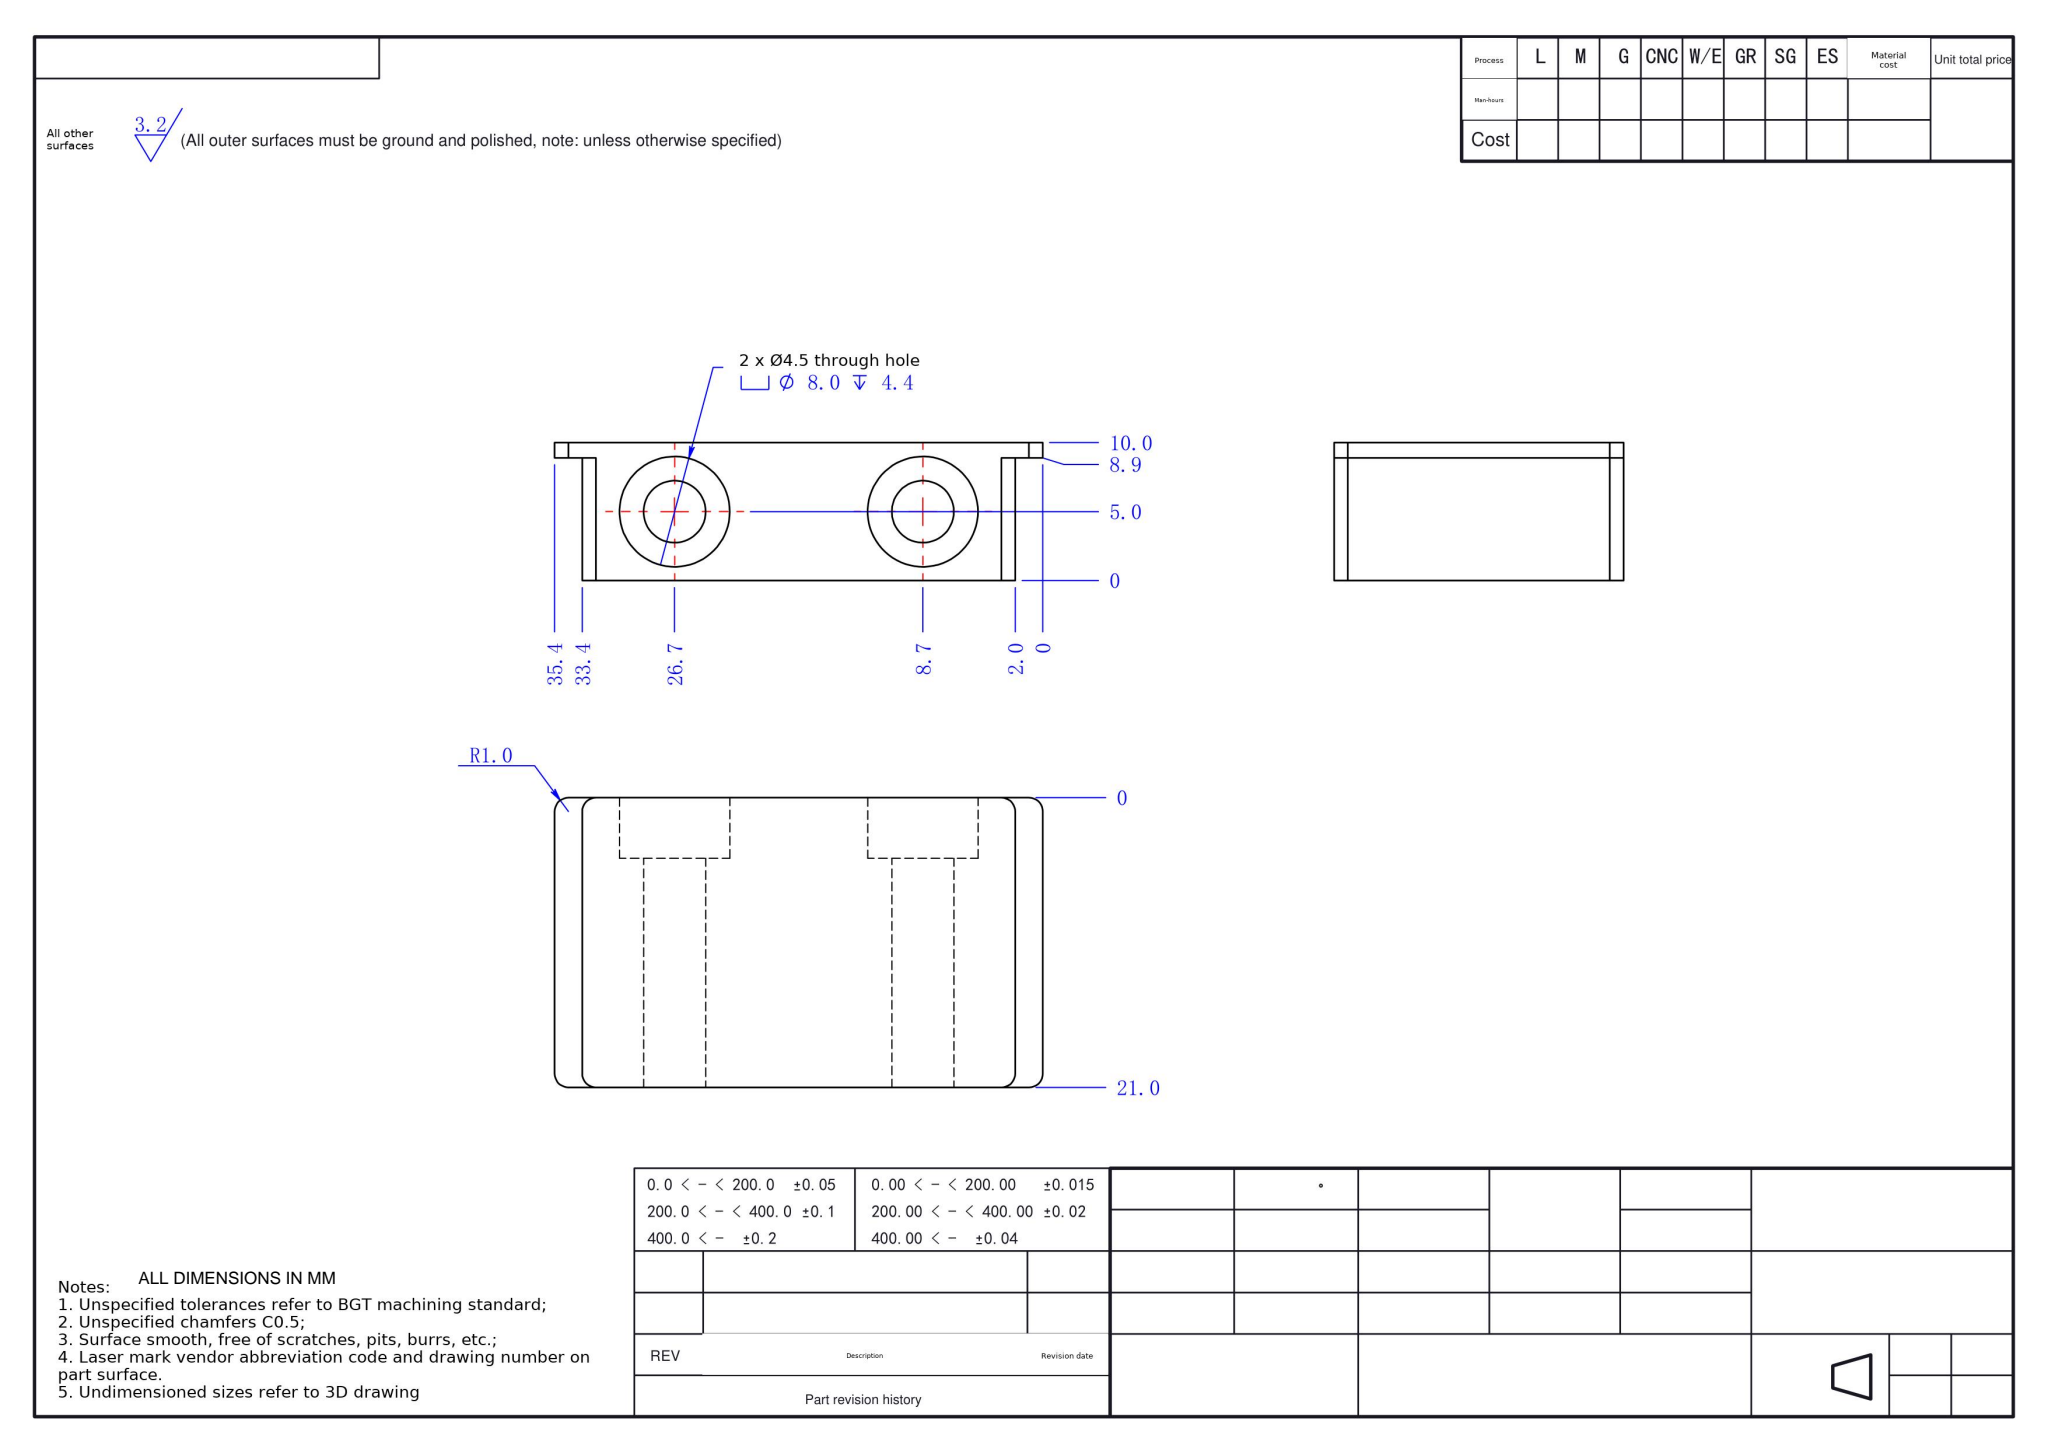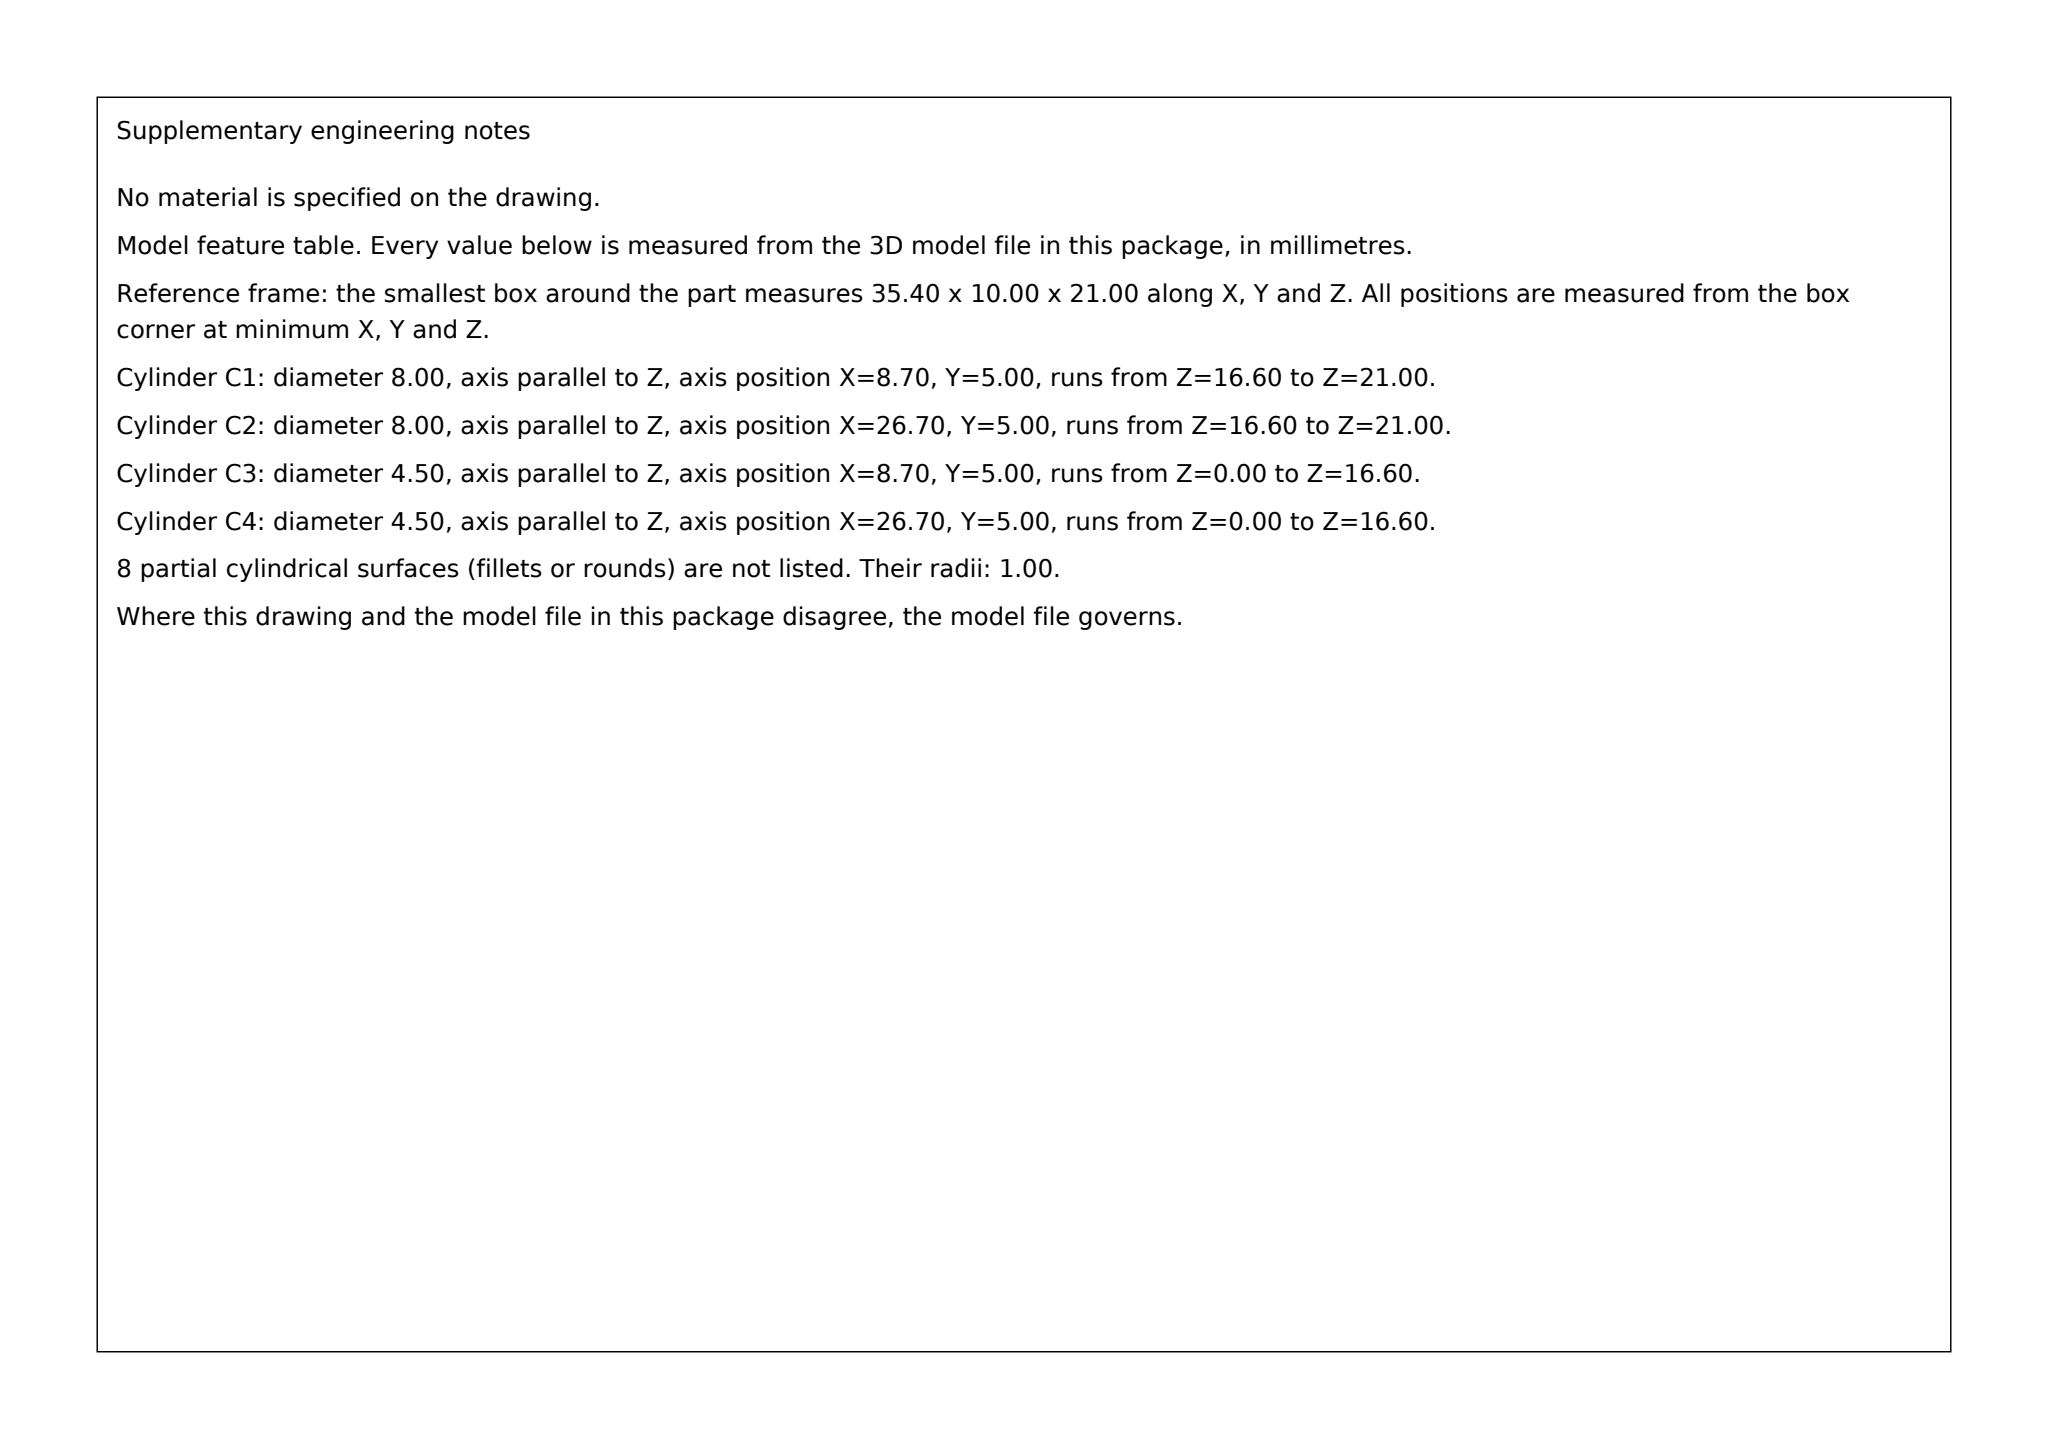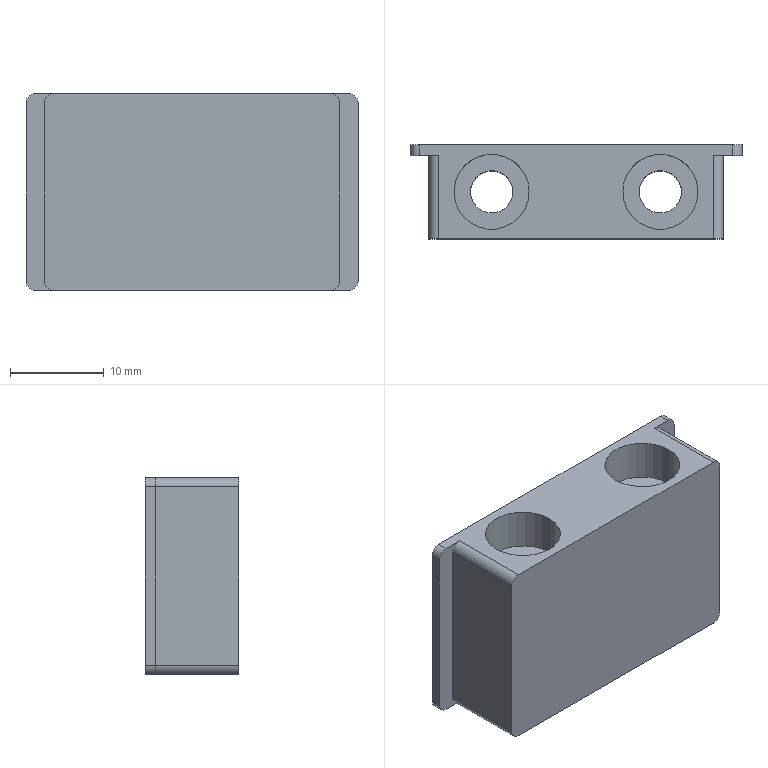Part | SolidWorks | mm | 1 solid | 28 faces | box 35.4 x 10 x 21 mm | volume 5707 mm3 | cylinder 16 | plane 12 | commonest cylinder face diameters 2 x8 8 x4 4.5 x4
build123d program:
from build123d import *

# Parameters (mm, degrees)
SKETCH1_W                                           = 35.4
SKETCH1_H                                           = 21
BOSS_EXTRUDE1_DEPTH                                 = 10
SKETCH2_W                                           = 2
SKETCH2_H                                           = 8.9
CUT_EXTRUDE1_DEPTH                                  = 30.228
SKETCH3_W                                           = 2
SKETCH3_H                                           = 8.9
CUT_EXTRUDE2_DEPTH                                  = 30.228
CYLINDRICAL_COUNTERSUNK_HOLE_FOR_M4_HEX_D           = 4.5
CYLINDRICAL_COUNTERSUNK_HOLE_FOR_M4_HEX_CBORE_D     = 8
CYLINDRICAL_COUNTERSUNK_HOLE_FOR_M4_HEX_CBORE_DEPTH = 4.4
FILLET1_R                                           = 1


with BuildPart() as part:
    # Sketch1 → Boss-Extrude1 (new body)
    with BuildSketch(Plane.XZ):
        with Locations((0, 10.5)):
            Rectangle(SKETCH1_W, SKETCH1_H)
    extrude(amount=-BOSS_EXTRUDE1_DEPTH)

    # Sketch2 → Cut-Extrude1 (cut, through all)
    with BuildSketch(Plane(origin=(0, 0, 0), x_dir=(-1, 0, 0), z_dir=(0, 0, -1))):
        with Locations((16.7, 4.45)):
            Rectangle(SKETCH2_W, SKETCH2_H)
    extrude(amount=-CUT_EXTRUDE1_DEPTH, mode=Mode.SUBTRACT)

    # Sketch3 → Cut-Extrude2 (cut, through all)
    with BuildSketch(Plane(origin=(0, 0, 0), x_dir=(-1, 0, 0), z_dir=(0, 0, -1))):
        with Locations((-16.7, 4.45)):
            Rectangle(SKETCH3_W, SKETCH3_H)
    extrude(amount=-CUT_EXTRUDE2_DEPTH, mode=Mode.SUBTRACT)

    # Cylindrical Countersunk Hole for M4 Hex (through all)
    with Locations(Plane.XY.offset(21)):
        with Locations((-9, 5), (9, 5)):
            CounterBoreHole(CYLINDRICAL_COUNTERSUNK_HOLE_FOR_M4_HEX_D / 2, CYLINDRICAL_COUNTERSUNK_HOLE_FOR_M4_HEX_CBORE_D / 2, CYLINDRICAL_COUNTERSUNK_HOLE_FOR_M4_HEX_CBORE_DEPTH)

    # Fillet1
    fillet1_edges = [part.edges().sort_by_distance(p)[0] for p in [
        (-15.7, 4.45, 21),
        (-15.7, 4.45, 0),
        (15.7, 4.45, 21),
        (15.7, 4.45, 0),
        (17.7, 9.45, 0),
        (-17.7, 9.45, 0),
        (-17.7, 9.45, 21),
        (17.7, 9.45, 21),
    ]]
    fillet(fillet1_edges, radius=FILLET1_R)


solid = part.part
STEP:
#1=CARTESIAN_POINT('',(-13.,5.,16.6));
#2=VERTEX_POINT('',#1);
#3=CARTESIAN_POINT('',(-5.,5.,16.6));
#4=VERTEX_POINT('',#3);
#5=CARTESIAN_POINT('',(-9.,5.,16.6));
#6=DIRECTION('',(0.,0.,1.));
#7=DIRECTION('',(1.,0.,0.));
#8=AXIS2_PLACEMENT_3D('',#5,#6,#7);
#9=CIRCLE('',#8,4.);
#10=EDGE_CURVE('',#2,#4,#9,.T.);
#11=ORIENTED_EDGE('',*,*,#10,.F.);
#12=CARTESIAN_POINT('',(-13.,5.,21.));
#13=VERTEX_POINT('',#12);
#14=CARTESIAN_POINT('',(-13.,5.,21.));
#15=DIRECTION('',(0.,0.,1.));
#16=VECTOR('',#15,1000.);
#17=LINE('',#14,#16);
#18=EDGE_CURVE('',#2,#13,#17,.T.);
#19=ORIENTED_EDGE('',*,*,#18,.T.);
#20=CARTESIAN_POINT('',(-5.,5.,21.));
#21=VERTEX_POINT('',#20);
#22=CARTESIAN_POINT('',(-9.,5.,21.));
#23=DIRECTION('',(0.,0.,1.));
#24=DIRECTION('',(1.,0.,0.));
#25=AXIS2_PLACEMENT_3D('',#22,#23,#24);
#26=CIRCLE('',#25,4.);
#27=EDGE_CURVE('',#13,#21,#26,.T.);
#28=ORIENTED_EDGE('',*,*,#27,.T.);
#29=CARTESIAN_POINT('',(-5.,5.,21.));
#30=DIRECTION('',(0.,0.,1.));
#31=VECTOR('',#30,1000.);
#32=LINE('',#29,#31);
#33=EDGE_CURVE('',#4,#21,#32,.T.);
#34=ORIENTED_EDGE('',*,*,#33,.F.);
#35=EDGE_LOOP('',(#11,#19,#28,#34));
#36=FACE_OUTER_BOUND('',#35,.T.);
#37=CARTESIAN_POINT('',(-9.,5.,21.));
#38=DIRECTION('',(0.,0.,1.));
#39=DIRECTION('',(1.,0.,0.));
#40=AXIS2_PLACEMENT_3D('',#37,#38,#39);
#41=CYLINDRICAL_SURFACE('',#40,4.);
#42=ADVANCED_FACE('',(#36),#41,.F.);
#43=CARTESIAN_POINT('',(-11.25,5.,-0.));
#44=VERTEX_POINT('',#43);
#45=CARTESIAN_POINT('',(-6.75,5.,-0.));
#46=VERTEX_POINT('',#45);
#47=CARTESIAN_POINT('',(-9.,5.,-0.));
#48=DIRECTION('',(0.,0.,1.));
#49=DIRECTION('',(1.,0.,0.));
#50=AXIS2_PLACEMENT_3D('',#47,#48,#49);
#51=CIRCLE('',#50,2.25);
#52=EDGE_CURVE('',#44,#46,#51,.T.);
#53=ORIENTED_EDGE('',*,*,#52,.F.);
#54=CARTESIAN_POINT('',(-11.25,5.,16.6));
#55=VERTEX_POINT('',#54);
#56=CARTESIAN_POINT('',(-11.25,5.,21.));
#57=DIRECTION('',(0.,0.,1.));
#58=VECTOR('',#57,1000.);
#59=LINE('',#56,#58);
#60=EDGE_CURVE('',#44,#55,#59,.T.);
#61=ORIENTED_EDGE('',*,*,#60,.T.);
#62=CARTESIAN_POINT('',(-6.75,5.,16.6));
#63=VERTEX_POINT('',#62);
#64=CARTESIAN_POINT('',(-9.,5.,16.6));
#65=DIRECTION('',(0.,0.,1.));
#66=DIRECTION('',(1.,0.,0.));
#67=AXIS2_PLACEMENT_3D('',#64,#65,#66);
#68=CIRCLE('',#67,2.25);
#69=EDGE_CURVE('',#55,#63,#68,.T.);
#70=ORIENTED_EDGE('',*,*,#69,.T.);
#71=CARTESIAN_POINT('',(-6.75,5.,21.));
#72=DIRECTION('',(0.,0.,1.));
#73=VECTOR('',#72,1000.);
#74=LINE('',#71,#73);
#75=EDGE_CURVE('',#46,#63,#74,.T.);
#76=ORIENTED_EDGE('',*,*,#75,.F.);
#77=EDGE_LOOP('',(#53,#61,#70,#76));
#78=FACE_OUTER_BOUND('',#77,.T.);
#79=CARTESIAN_POINT('',(-9.,5.,21.));
#80=DIRECTION('',(0.,0.,1.));
#81=DIRECTION('',(1.,0.,0.));
#82=AXIS2_PLACEMENT_3D('',#79,#80,#81);
#83=CYLINDRICAL_SURFACE('',#82,2.25);
#84=ADVANCED_FACE('',(#78),#83,.F.);
#85=CARTESIAN_POINT('',(5.,5.,16.6));
#86=VERTEX_POINT('',#85);
#87=CARTESIAN_POINT('',(13.,5.,16.6));
#88=VERTEX_POINT('',#87);
#89=CARTESIAN_POINT('',(9.,5.,16.6));
#90=DIRECTION('',(0.,0.,1.));
#91=DIRECTION('',(1.,0.,0.));
#92=AXIS2_PLACEMENT_3D('',#89,#90,#91);
#93=CIRCLE('',#92,4.);
#94=EDGE_CURVE('',#86,#88,#93,.T.);
#95=ORIENTED_EDGE('',*,*,#94,.F.);
#96=CARTESIAN_POINT('',(5.,5.,21.));
#97=VERTEX_POINT('',#96);
#98=CARTESIAN_POINT('',(5.,5.,21.));
#99=DIRECTION('',(0.,0.,1.));
#100=VECTOR('',#99,1000.);
#101=LINE('',#98,#100);
#102=EDGE_CURVE('',#86,#97,#101,.T.);
#103=ORIENTED_EDGE('',*,*,#102,.T.);
#104=CARTESIAN_POINT('',(13.,5.,21.));
#105=VERTEX_POINT('',#104);
#106=CARTESIAN_POINT('',(9.,5.,21.));
#107=DIRECTION('',(0.,0.,1.));
#108=DIRECTION('',(1.,0.,0.));
#109=AXIS2_PLACEMENT_3D('',#106,#107,#108);
#110=CIRCLE('',#109,4.);
#111=EDGE_CURVE('',#97,#105,#110,.T.);
#112=ORIENTED_EDGE('',*,*,#111,.T.);
#113=CARTESIAN_POINT('',(13.,5.,21.));
#114=DIRECTION('',(0.,0.,1.));
#115=VECTOR('',#114,1000.);
#116=LINE('',#113,#115);
#117=EDGE_CURVE('',#88,#105,#116,.T.);
#118=ORIENTED_EDGE('',*,*,#117,.F.);
#119=EDGE_LOOP('',(#95,#103,#112,#118));
#120=FACE_OUTER_BOUND('',#119,.T.);
#121=CARTESIAN_POINT('',(9.,5.,21.));
#122=DIRECTION('',(0.,0.,1.));
#123=DIRECTION('',(1.,0.,0.));
#124=AXIS2_PLACEMENT_3D('',#121,#122,#123);
#125=CYLINDRICAL_SURFACE('',#124,4.);
#126=ADVANCED_FACE('',(#120),#125,.F.);
#127=CARTESIAN_POINT('',(6.75,5.,-0.));
#128=VERTEX_POINT('',#127);
#129=CARTESIAN_POINT('',(11.25,5.,-0.));
#130=VERTEX_POINT('',#129);
#131=CARTESIAN_POINT('',(9.,5.,-0.));
#132=DIRECTION('',(0.,0.,1.));
#133=DIRECTION('',(1.,0.,0.));
#134=AXIS2_PLACEMENT_3D('',#131,#132,#133);
#135=CIRCLE('',#134,2.25);
#136=EDGE_CURVE('',#128,#130,#135,.T.);
#137=ORIENTED_EDGE('',*,*,#136,.F.);
#138=CARTESIAN_POINT('',(6.75,5.,16.6));
#139=VERTEX_POINT('',#138);
#140=CARTESIAN_POINT('',(6.75,5.,21.));
#141=DIRECTION('',(0.,0.,1.));
#142=VECTOR('',#141,1000.);
#143=LINE('',#140,#142);
#144=EDGE_CURVE('',#128,#139,#143,.T.);
#145=ORIENTED_EDGE('',*,*,#144,.T.);
#146=CARTESIAN_POINT('',(11.25,5.,16.6));
#147=VERTEX_POINT('',#146);
#148=CARTESIAN_POINT('',(9.,5.,16.6));
#149=DIRECTION('',(0.,0.,1.));
#150=DIRECTION('',(1.,0.,0.));
#151=AXIS2_PLACEMENT_3D('',#148,#149,#150);
#152=CIRCLE('',#151,2.25);
#153=EDGE_CURVE('',#139,#147,#152,.T.);
#154=ORIENTED_EDGE('',*,*,#153,.T.);
#155=CARTESIAN_POINT('',(11.25,5.,21.));
#156=DIRECTION('',(0.,0.,1.));
#157=VECTOR('',#156,1000.);
#158=LINE('',#155,#157);
#159=EDGE_CURVE('',#130,#147,#158,.T.);
#160=ORIENTED_EDGE('',*,*,#159,.F.);
#161=EDGE_LOOP('',(#137,#145,#154,#160));
#162=FACE_OUTER_BOUND('',#161,.T.);
#163=CARTESIAN_POINT('',(9.,5.,21.));
#164=DIRECTION('',(0.,0.,1.));
#165=DIRECTION('',(1.,0.,0.));
#166=AXIS2_PLACEMENT_3D('',#163,#164,#165);
#167=CYLINDRICAL_SURFACE('',#166,2.25);
#168=ADVANCED_FACE('',(#162),#167,.F.);
#169=CARTESIAN_POINT('',(17.7,8.9,20.));
#170=VERTEX_POINT('',#169);
#171=CARTESIAN_POINT('',(17.7,8.9,1.));
#172=VERTEX_POINT('',#171);
#173=CARTESIAN_POINT('',(17.7,8.9,21.));
#174=DIRECTION('',(0.,0.,-1.));
#175=VECTOR('',#174,1000.);
#176=LINE('',#173,#175);
#177=EDGE_CURVE('',#170,#172,#176,.T.);
#178=ORIENTED_EDGE('',*,*,#177,.T.);
#179=CARTESIAN_POINT('',(17.7,10.,1.));
#180=VERTEX_POINT('',#179);
#181=CARTESIAN_POINT('',(17.7,10.,1.));
#182=DIRECTION('',(0.,1.,0.));
#183=VECTOR('',#182,1000.);
#184=LINE('',#181,#183);
#185=EDGE_CURVE('',#172,#180,#184,.T.);
#186=ORIENTED_EDGE('',*,*,#185,.T.);
#187=CARTESIAN_POINT('',(17.7,10.,20.));
#188=VERTEX_POINT('',#187);
#189=CARTESIAN_POINT('',(17.7,10.,0.));
#190=DIRECTION('',(0.,0.,1.));
#191=VECTOR('',#190,1000.);
#192=LINE('',#189,#191);
#193=EDGE_CURVE('',#180,#188,#192,.T.);
#194=ORIENTED_EDGE('',*,*,#193,.T.);
#195=CARTESIAN_POINT('',(17.7,10.,20.));
#196=DIRECTION('',(0.,-1.,0.));
#197=VECTOR('',#196,1000.);
#198=LINE('',#195,#197);
#199=EDGE_CURVE('',#188,#170,#198,.T.);
#200=ORIENTED_EDGE('',*,*,#199,.T.);
#201=EDGE_LOOP('',(#178,#186,#194,#200));
#202=FACE_OUTER_BOUND('',#201,.T.);
#203=CARTESIAN_POINT('',(17.7,10.,0.));
#204=DIRECTION('',(1.,0.,0.));
#205=DIRECTION('',(0.,0.,-1.));
#206=AXIS2_PLACEMENT_3D('',#203,#204,#205);
#207=PLANE('',#206);
#208=ADVANCED_FACE('',(#202),#207,.T.);
#209=CARTESIAN_POINT('',(-9.,5.,-0.));
#210=DIRECTION('',(0.,0.,1.));
#211=DIRECTION('',(1.,0.,0.));
#212=AXIS2_PLACEMENT_3D('',#209,#210,#211);
#213=CIRCLE('',#212,2.25);
#214=EDGE_CURVE('',#46,#44,#213,.T.);
#215=ORIENTED_EDGE('',*,*,#214,.T.);
#216=ORIENTED_EDGE('',*,*,#52,.T.);
#217=EDGE_LOOP('',(#215,#216));
#218=FACE_BOUND('',#217,.T.);
#219=CARTESIAN_POINT('',(9.,5.,-0.));
#220=DIRECTION('',(0.,0.,1.));
#221=DIRECTION('',(1.,0.,0.));
#222=AXIS2_PLACEMENT_3D('',#219,#220,#221);
#223=CIRCLE('',#222,2.25);
#224=EDGE_CURVE('',#130,#128,#223,.T.);
#225=ORIENTED_EDGE('',*,*,#224,.T.);
#226=ORIENTED_EDGE('',*,*,#136,.T.);
#227=EDGE_LOOP('',(#225,#226));
#228=FACE_BOUND('',#227,.T.);
#229=CARTESIAN_POINT('',(-16.7,10.,0.));
#230=VERTEX_POINT('',#229);
#231=CARTESIAN_POINT('',(16.7,10.,0.));
#232=VERTEX_POINT('',#231);
#233=CARTESIAN_POINT('',(-17.7,10.,0.));
#234=DIRECTION('',(1.,0.,0.));
#235=VECTOR('',#234,1000.);
#236=LINE('',#233,#235);
#237=EDGE_CURVE('',#230,#232,#236,.T.);
#238=ORIENTED_EDGE('',*,*,#237,.T.);
#239=CARTESIAN_POINT('',(16.7,8.9,0.));
#240=VERTEX_POINT('',#239);
#241=CARTESIAN_POINT('',(16.7,10.,0.));
#242=DIRECTION('',(0.,-1.,0.));
#243=VECTOR('',#242,1000.);
#244=LINE('',#241,#243);
#245=EDGE_CURVE('',#232,#240,#244,.T.);
#246=ORIENTED_EDGE('',*,*,#245,.T.);
#247=CARTESIAN_POINT('',(14.7,8.9,0.));
#248=VERTEX_POINT('',#247);
#249=CARTESIAN_POINT('',(15.7,8.9,0.));
#250=DIRECTION('',(1.,0.,0.));
#251=VECTOR('',#250,1000.);
#252=LINE('',#249,#251);
#253=EDGE_CURVE('',#248,#240,#252,.T.);
#254=ORIENTED_EDGE('',*,*,#253,.F.);
#255=CARTESIAN_POINT('',(14.7,0.,0.));
#256=VERTEX_POINT('',#255);
#257=CARTESIAN_POINT('',(14.7,0.,0.));
#258=DIRECTION('',(0.,-1.,0.));
#259=VECTOR('',#258,1000.);
#260=LINE('',#257,#259);
#261=EDGE_CURVE('',#248,#256,#260,.T.);
#262=ORIENTED_EDGE('',*,*,#261,.T.);
#263=CARTESIAN_POINT('',(-14.7,0.,0.));
#264=VERTEX_POINT('',#263);
#265=CARTESIAN_POINT('',(-17.7,0.,0.));
#266=DIRECTION('',(1.,0.,0.));
#267=VECTOR('',#266,1000.);
#268=LINE('',#265,#267);
#269=EDGE_CURVE('',#264,#256,#268,.T.);
#270=ORIENTED_EDGE('',*,*,#269,.F.);
#271=CARTESIAN_POINT('',(-14.7,8.9,0.));
#272=VERTEX_POINT('',#271);
#273=CARTESIAN_POINT('',(-14.7,8.9,0.));
#274=DIRECTION('',(0.,1.,0.));
#275=VECTOR('',#274,1000.);
#276=LINE('',#273,#275);
#277=EDGE_CURVE('',#264,#272,#276,.T.);
#278=ORIENTED_EDGE('',*,*,#277,.T.);
#279=CARTESIAN_POINT('',(-16.7,8.9,0.));
#280=VERTEX_POINT('',#279);
#281=CARTESIAN_POINT('',(-17.7,8.9,0.));
#282=DIRECTION('',(1.,0.,0.));
#283=VECTOR('',#282,1000.);
#284=LINE('',#281,#283);
#285=EDGE_CURVE('',#280,#272,#284,.T.);
#286=ORIENTED_EDGE('',*,*,#285,.F.);
#287=CARTESIAN_POINT('',(-16.7,10.,0.));
#288=DIRECTION('',(0.,1.,0.));
#289=VECTOR('',#288,1000.);
#290=LINE('',#287,#289);
#291=EDGE_CURVE('',#280,#230,#290,.T.);
#292=ORIENTED_EDGE('',*,*,#291,.T.);
#293=EDGE_LOOP('',(#238,#246,#254,#262,#270,#278,#286,#292));
#294=FACE_OUTER_BOUND('',#293,.T.);
#295=CARTESIAN_POINT('',(-17.7,10.,0.));
#296=DIRECTION('',(0.,0.,-1.));
#297=DIRECTION('',(-1.,0.,0.));
#298=AXIS2_PLACEMENT_3D('',#295,#296,#297);
#299=PLANE('',#298);
#300=ADVANCED_FACE('',(#218,#228,#294),#299,.T.);
#301=CARTESIAN_POINT('',(-17.7,8.9,20.));
#302=VERTEX_POINT('',#301);
#303=CARTESIAN_POINT('',(-17.7,8.9,1.));
#304=VERTEX_POINT('',#303);
#305=CARTESIAN_POINT('',(-17.7,8.9,21.));
#306=DIRECTION('',(0.,0.,-1.));
#307=VECTOR('',#306,1000.);
#308=LINE('',#305,#307);
#309=EDGE_CURVE('',#302,#304,#308,.T.);
#310=ORIENTED_EDGE('',*,*,#309,.F.);
#311=CARTESIAN_POINT('',(-17.7,10.,20.));
#312=VERTEX_POINT('',#311);
#313=CARTESIAN_POINT('',(-17.7,10.,20.));
#314=DIRECTION('',(0.,1.,0.));
#315=VECTOR('',#314,1000.);
#316=LINE('',#313,#315);
#317=EDGE_CURVE('',#302,#312,#316,.T.);
#318=ORIENTED_EDGE('',*,*,#317,.T.);
#319=CARTESIAN_POINT('',(-17.7,10.,1.));
#320=VERTEX_POINT('',#319);
#321=CARTESIAN_POINT('',(-17.7,10.,21.));
#322=DIRECTION('',(0.,0.,-1.));
#323=VECTOR('',#322,1000.);
#324=LINE('',#321,#323);
#325=EDGE_CURVE('',#312,#320,#324,.T.);
#326=ORIENTED_EDGE('',*,*,#325,.T.);
#327=CARTESIAN_POINT('',(-17.7,10.,1.));
#328=DIRECTION('',(0.,-1.,0.));
#329=VECTOR('',#328,1000.);
#330=LINE('',#327,#329);
#331=EDGE_CURVE('',#320,#304,#330,.T.);
#332=ORIENTED_EDGE('',*,*,#331,.T.);
#333=EDGE_LOOP('',(#310,#318,#326,#332));
#334=FACE_OUTER_BOUND('',#333,.T.);
#335=CARTESIAN_POINT('',(-17.7,10.,21.));
#336=DIRECTION('',(-1.,0.,0.));
#337=DIRECTION('',(0.,0.,1.));
#338=AXIS2_PLACEMENT_3D('',#335,#336,#337);
#339=PLANE('',#338);
#340=ADVANCED_FACE('',(#334),#339,.T.);
#341=CARTESIAN_POINT('',(-9.,5.,21.));
#342=DIRECTION('',(0.,0.,1.));
#343=DIRECTION('',(1.,0.,0.));
#344=AXIS2_PLACEMENT_3D('',#341,#342,#343);
#345=CIRCLE('',#344,4.);
#346=EDGE_CURVE('',#21,#13,#345,.T.);
#347=ORIENTED_EDGE('',*,*,#346,.F.);
#348=ORIENTED_EDGE('',*,*,#27,.F.);
#349=EDGE_LOOP('',(#347,#348));
#350=FACE_BOUND('',#349,.T.);
#351=CARTESIAN_POINT('',(9.,5.,21.));
#352=DIRECTION('',(0.,0.,1.));
#353=DIRECTION('',(1.,0.,0.));
#354=AXIS2_PLACEMENT_3D('',#351,#352,#353);
#355=CIRCLE('',#354,4.);
#356=EDGE_CURVE('',#105,#97,#355,.T.);
#357=ORIENTED_EDGE('',*,*,#356,.F.);
#358=ORIENTED_EDGE('',*,*,#111,.F.);
#359=EDGE_LOOP('',(#357,#358));
#360=FACE_BOUND('',#359,.T.);
#361=CARTESIAN_POINT('',(16.7,10.,21.));
#362=VERTEX_POINT('',#361);
#363=CARTESIAN_POINT('',(-16.7,10.,21.));
#364=VERTEX_POINT('',#363);
#365=CARTESIAN_POINT('',(17.7,10.,21.));
#366=DIRECTION('',(-1.,0.,0.));
#367=VECTOR('',#366,1000.);
#368=LINE('',#365,#367);
#369=EDGE_CURVE('',#362,#364,#368,.T.);
#370=ORIENTED_EDGE('',*,*,#369,.T.);
#371=CARTESIAN_POINT('',(-16.7,8.9,21.));
#372=VERTEX_POINT('',#371);
#373=CARTESIAN_POINT('',(-16.7,10.,21.));
#374=DIRECTION('',(0.,-1.,0.));
#375=VECTOR('',#374,1000.);
#376=LINE('',#373,#375);
#377=EDGE_CURVE('',#364,#372,#376,.T.);
#378=ORIENTED_EDGE('',*,*,#377,.T.);
#379=CARTESIAN_POINT('',(-14.7,8.9,21.));
#380=VERTEX_POINT('',#379);
#381=CARTESIAN_POINT('',(-17.7,8.9,21.));
#382=DIRECTION('',(1.,0.,0.));
#383=VECTOR('',#382,1000.);
#384=LINE('',#381,#383);
#385=EDGE_CURVE('',#372,#380,#384,.T.);
#386=ORIENTED_EDGE('',*,*,#385,.T.);
#387=CARTESIAN_POINT('',(-14.7,0.,21.));
#388=VERTEX_POINT('',#387);
#389=CARTESIAN_POINT('',(-14.7,0.,21.));
#390=DIRECTION('',(0.,-1.,0.));
#391=VECTOR('',#390,1000.);
#392=LINE('',#389,#391);
#393=EDGE_CURVE('',#380,#388,#392,.T.);
#394=ORIENTED_EDGE('',*,*,#393,.T.);
#395=CARTESIAN_POINT('',(14.7,0.,21.));
#396=VERTEX_POINT('',#395);
#397=CARTESIAN_POINT('',(17.7,0.,21.));
#398=DIRECTION('',(-1.,0.,0.));
#399=VECTOR('',#398,1000.);
#400=LINE('',#397,#399);
#401=EDGE_CURVE('',#396,#388,#400,.T.);
#402=ORIENTED_EDGE('',*,*,#401,.F.);
#403=CARTESIAN_POINT('',(14.7,8.9,21.));
#404=VERTEX_POINT('',#403);
#405=CARTESIAN_POINT('',(14.7,8.9,21.));
#406=DIRECTION('',(0.,1.,0.));
#407=VECTOR('',#406,1000.);
#408=LINE('',#405,#407);
#409=EDGE_CURVE('',#396,#404,#408,.T.);
#410=ORIENTED_EDGE('',*,*,#409,.T.);
#411=CARTESIAN_POINT('',(16.7,8.9,21.));
#412=VERTEX_POINT('',#411);
#413=CARTESIAN_POINT('',(15.7,8.9,21.));
#414=DIRECTION('',(1.,0.,0.));
#415=VECTOR('',#414,1000.);
#416=LINE('',#413,#415);
#417=EDGE_CURVE('',#404,#412,#416,.T.);
#418=ORIENTED_EDGE('',*,*,#417,.T.);
#419=CARTESIAN_POINT('',(16.7,10.,21.));
#420=DIRECTION('',(0.,1.,0.));
#421=VECTOR('',#420,1000.);
#422=LINE('',#419,#421);
#423=EDGE_CURVE('',#412,#362,#422,.T.);
#424=ORIENTED_EDGE('',*,*,#423,.T.);
#425=EDGE_LOOP('',(#370,#378,#386,#394,#402,#410,#418,#424));
#426=FACE_OUTER_BOUND('',#425,.T.);
#427=CARTESIAN_POINT('',(17.7,10.,21.));
#428=DIRECTION('',(0.,0.,1.));
#429=DIRECTION('',(1.,0.,0.));
#430=AXIS2_PLACEMENT_3D('',#427,#428,#429);
#431=PLANE('',#430);
#432=ADVANCED_FACE('',(#350,#360,#426),#431,.T.);
#433=ORIENTED_EDGE('',*,*,#193,.F.);
#434=CARTESIAN_POINT('',(16.7,10.,1.));
#435=DIRECTION('',(0.,1.,0.));
#436=DIRECTION('',(-0.,0.,-1.));
#437=AXIS2_PLACEMENT_3D('',#434,#435,#436);
#438=CIRCLE('',#437,1.);
#439=EDGE_CURVE('',#180,#232,#438,.T.);
#440=ORIENTED_EDGE('',*,*,#439,.T.);
#441=ORIENTED_EDGE('',*,*,#237,.F.);
#442=CARTESIAN_POINT('',(-16.7,10.,1.));
#443=DIRECTION('',(0.,1.,0.));
#444=DIRECTION('',(0.,0.,-1.));
#445=AXIS2_PLACEMENT_3D('',#442,#443,#444);
#446=CIRCLE('',#445,1.);
#447=EDGE_CURVE('',#230,#320,#446,.T.);
#448=ORIENTED_EDGE('',*,*,#447,.T.);
#449=ORIENTED_EDGE('',*,*,#325,.F.);
#450=CARTESIAN_POINT('',(-16.7,10.,20.));
#451=DIRECTION('',(0.,1.,0.));
#452=DIRECTION('',(0.,0.,-1.));
#453=AXIS2_PLACEMENT_3D('',#450,#451,#452);
#454=CIRCLE('',#453,1.);
#455=EDGE_CURVE('',#312,#364,#454,.T.);
#456=ORIENTED_EDGE('',*,*,#455,.T.);
#457=ORIENTED_EDGE('',*,*,#369,.F.);
#458=CARTESIAN_POINT('',(16.7,10.,20.));
#459=DIRECTION('',(0.,1.,0.));
#460=DIRECTION('',(0.,0.,-1.));
#461=AXIS2_PLACEMENT_3D('',#458,#459,#460);
#462=CIRCLE('',#461,1.);
#463=EDGE_CURVE('',#362,#188,#462,.T.);
#464=ORIENTED_EDGE('',*,*,#463,.T.);
#465=EDGE_LOOP('',(#433,#440,#441,#448,#449,#456,#457,#464));
#466=FACE_OUTER_BOUND('',#465,.T.);
#467=CARTESIAN_POINT('',(0.,10.,0.));
#468=DIRECTION('',(0.,-1.,0.));
#469=DIRECTION('',(0.,0.,-1.));
#470=AXIS2_PLACEMENT_3D('',#467,#468,#469);
#471=PLANE('',#470);
#472=ADVANCED_FACE('',(#466),#471,.F.);
#473=CARTESIAN_POINT('',(15.7,0.,20.));
#474=VERTEX_POINT('',#473);
#475=CARTESIAN_POINT('',(15.7,0.,1.));
#476=VERTEX_POINT('',#475);
#477=CARTESIAN_POINT('',(15.7,0.,21.));
#478=DIRECTION('',(0.,0.,-1.));
#479=VECTOR('',#478,1000.);
#480=LINE('',#477,#479);
#481=EDGE_CURVE('',#474,#476,#480,.T.);
#482=ORIENTED_EDGE('',*,*,#481,.F.);
#483=CARTESIAN_POINT('',(14.7,0.,20.));
#484=DIRECTION('',(0.,-1.,0.));
#485=DIRECTION('',(0.,0.,-1.));
#486=AXIS2_PLACEMENT_3D('',#483,#484,#485);
#487=CIRCLE('',#486,1.);
#488=EDGE_CURVE('',#474,#396,#487,.T.);
#489=ORIENTED_EDGE('',*,*,#488,.T.);
#490=ORIENTED_EDGE('',*,*,#401,.T.);
#491=CARTESIAN_POINT('',(-15.7,0.,20.));
#492=VERTEX_POINT('',#491);
#493=CARTESIAN_POINT('',(-14.7,0.,20.));
#494=DIRECTION('',(0.,-1.,0.));
#495=DIRECTION('',(0.,0.,-1.));
#496=AXIS2_PLACEMENT_3D('',#493,#494,#495);
#497=CIRCLE('',#496,1.);
#498=EDGE_CURVE('',#388,#492,#497,.T.);
#499=ORIENTED_EDGE('',*,*,#498,.T.);
#500=CARTESIAN_POINT('',(-15.7,0.,1.));
#501=VERTEX_POINT('',#500);
#502=CARTESIAN_POINT('',(-15.7,0.,21.));
#503=DIRECTION('',(0.,0.,-1.));
#504=VECTOR('',#503,1000.);
#505=LINE('',#502,#504);
#506=EDGE_CURVE('',#492,#501,#505,.T.);
#507=ORIENTED_EDGE('',*,*,#506,.T.);
#508=CARTESIAN_POINT('',(-14.7,0.,1.));
#509=DIRECTION('',(0.,-1.,0.));
#510=DIRECTION('',(0.,0.,-1.));
#511=AXIS2_PLACEMENT_3D('',#508,#509,#510);
#512=CIRCLE('',#511,1.);
#513=EDGE_CURVE('',#501,#264,#512,.T.);
#514=ORIENTED_EDGE('',*,*,#513,.T.);
#515=ORIENTED_EDGE('',*,*,#269,.T.);
#516=CARTESIAN_POINT('',(14.7,0.,1.));
#517=DIRECTION('',(0.,-1.,0.));
#518=DIRECTION('',(0.,0.,-1.));
#519=AXIS2_PLACEMENT_3D('',#516,#517,#518);
#520=CIRCLE('',#519,1.);
#521=EDGE_CURVE('',#256,#476,#520,.T.);
#522=ORIENTED_EDGE('',*,*,#521,.T.);
#523=EDGE_LOOP('',(#482,#489,#490,#499,#507,#514,#515,#522));
#524=FACE_OUTER_BOUND('',#523,.T.);
#525=CARTESIAN_POINT('',(0.,0.,0.));
#526=DIRECTION('',(0.,-1.,0.));
#527=DIRECTION('',(0.,0.,-1.));
#528=AXIS2_PLACEMENT_3D('',#525,#526,#527);
#529=PLANE('',#528);
#530=ADVANCED_FACE('',(#524),#529,.T.);
#531=ORIENTED_EDGE('',*,*,#385,.F.);
#532=CARTESIAN_POINT('',(-16.7,8.9,20.));
#533=DIRECTION('',(0.,-1.,0.));
#534=DIRECTION('',(0.,0.,1.));
#535=AXIS2_PLACEMENT_3D('',#532,#533,#534);
#536=CIRCLE('',#535,1.);
#537=EDGE_CURVE('',#372,#302,#536,.T.);
#538=ORIENTED_EDGE('',*,*,#537,.T.);
#539=ORIENTED_EDGE('',*,*,#309,.T.);
#540=CARTESIAN_POINT('',(-16.7,8.9,1.));
#541=DIRECTION('',(0.,-1.,0.));
#542=DIRECTION('',(0.,0.,1.));
#543=AXIS2_PLACEMENT_3D('',#540,#541,#542);
#544=CIRCLE('',#543,1.);
#545=EDGE_CURVE('',#304,#280,#544,.T.);
#546=ORIENTED_EDGE('',*,*,#545,.T.);
#547=ORIENTED_EDGE('',*,*,#285,.T.);
#548=CARTESIAN_POINT('',(-15.7,8.9,1.));
#549=VERTEX_POINT('',#548);
#550=CARTESIAN_POINT('',(-14.7,8.9,1.));
#551=DIRECTION('',(0.,1.,0.));
#552=DIRECTION('',(0.,0.,1.));
#553=AXIS2_PLACEMENT_3D('',#550,#551,#552);
#554=CIRCLE('',#553,1.);
#555=EDGE_CURVE('',#272,#549,#554,.T.);
#556=ORIENTED_EDGE('',*,*,#555,.T.);
#557=CARTESIAN_POINT('',(-15.7,8.9,20.));
#558=VERTEX_POINT('',#557);
#559=CARTESIAN_POINT('',(-15.7,8.9,21.));
#560=DIRECTION('',(0.,0.,-1.));
#561=VECTOR('',#560,1000.);
#562=LINE('',#559,#561);
#563=EDGE_CURVE('',#558,#549,#562,.T.);
#564=ORIENTED_EDGE('',*,*,#563,.F.);
#565=CARTESIAN_POINT('',(-14.7,8.9,20.));
#566=DIRECTION('',(0.,1.,0.));
#567=DIRECTION('',(0.,0.,1.));
#568=AXIS2_PLACEMENT_3D('',#565,#566,#567);
#569=CIRCLE('',#568,1.);
#570=EDGE_CURVE('',#558,#380,#569,.T.);
#571=ORIENTED_EDGE('',*,*,#570,.T.);
#572=EDGE_LOOP('',(#531,#538,#539,#546,#547,#556,#564,#571));
#573=FACE_OUTER_BOUND('',#572,.T.);
#574=CARTESIAN_POINT('',(-17.7,8.9,21.));
#575=DIRECTION('',(0.,1.,0.));
#576=DIRECTION('',(0.,0.,1.));
#577=AXIS2_PLACEMENT_3D('',#574,#575,#576);
#578=PLANE('',#577);
#579=ADVANCED_FACE('',(#573),#578,.F.);
#580=ORIENTED_EDGE('',*,*,#563,.T.);
#581=CARTESIAN_POINT('',(-15.7,0.,1.));
#582=DIRECTION('',(0.,-1.,0.));
#583=VECTOR('',#582,1000.);
#584=LINE('',#581,#583);
#585=EDGE_CURVE('',#549,#501,#584,.T.);
#586=ORIENTED_EDGE('',*,*,#585,.T.);
#587=ORIENTED_EDGE('',*,*,#506,.F.);
#588=CARTESIAN_POINT('',(-15.7,8.9,20.));
#589=DIRECTION('',(0.,1.,0.));
#590=VECTOR('',#589,1000.);
#591=LINE('',#588,#590);
#592=EDGE_CURVE('',#492,#558,#591,.T.);
#593=ORIENTED_EDGE('',*,*,#592,.T.);
#594=EDGE_LOOP('',(#580,#586,#587,#593));
#595=FACE_OUTER_BOUND('',#594,.T.);
#596=CARTESIAN_POINT('',(-15.7,8.9,21.));
#597=DIRECTION('',(1.,0.,0.));
#598=DIRECTION('',(0.,0.,-1.));
#599=AXIS2_PLACEMENT_3D('',#596,#597,#598);
#600=PLANE('',#599);
#601=ADVANCED_FACE('',(#595),#600,.F.);
#602=ORIENTED_EDGE('',*,*,#253,.T.);
#603=CARTESIAN_POINT('',(16.7,8.9,1.));
#604=DIRECTION('',(0.,-1.,0.));
#605=DIRECTION('',(0.,0.,1.));
#606=AXIS2_PLACEMENT_3D('',#603,#604,#605);
#607=CIRCLE('',#606,1.);
#608=EDGE_CURVE('',#240,#172,#607,.T.);
#609=ORIENTED_EDGE('',*,*,#608,.T.);
#610=ORIENTED_EDGE('',*,*,#177,.F.);
#611=CARTESIAN_POINT('',(16.7,8.9,20.));
#612=DIRECTION('',(0.,-1.,0.));
#613=DIRECTION('',(0.,0.,1.));
#614=AXIS2_PLACEMENT_3D('',#611,#612,#613);
#615=CIRCLE('',#614,1.);
#616=EDGE_CURVE('',#170,#412,#615,.T.);
#617=ORIENTED_EDGE('',*,*,#616,.T.);
#618=ORIENTED_EDGE('',*,*,#417,.F.);
#619=CARTESIAN_POINT('',(15.7,8.9,20.));
#620=VERTEX_POINT('',#619);
#621=CARTESIAN_POINT('',(14.7,8.9,20.));
#622=DIRECTION('',(0.,1.,0.));
#623=DIRECTION('',(0.,0.,1.));
#624=AXIS2_PLACEMENT_3D('',#621,#622,#623);
#625=CIRCLE('',#624,1.);
#626=EDGE_CURVE('',#404,#620,#625,.T.);
#627=ORIENTED_EDGE('',*,*,#626,.T.);
#628=CARTESIAN_POINT('',(15.7,8.9,1.));
#629=VERTEX_POINT('',#628);
#630=CARTESIAN_POINT('',(15.7,8.9,21.));
#631=DIRECTION('',(0.,0.,-1.));
#632=VECTOR('',#631,1000.);
#633=LINE('',#630,#632);
#634=EDGE_CURVE('',#620,#629,#633,.T.);
#635=ORIENTED_EDGE('',*,*,#634,.T.);
#636=CARTESIAN_POINT('',(14.7,8.9,1.));
#637=DIRECTION('',(0.,1.,0.));
#638=DIRECTION('',(0.,0.,1.));
#639=AXIS2_PLACEMENT_3D('',#636,#637,#638);
#640=CIRCLE('',#639,1.);
#641=EDGE_CURVE('',#629,#248,#640,.T.);
#642=ORIENTED_EDGE('',*,*,#641,.T.);
#643=EDGE_LOOP('',(#602,#609,#610,#617,#618,#627,#635,#642));
#644=FACE_OUTER_BOUND('',#643,.T.);
#645=CARTESIAN_POINT('',(15.7,8.9,21.));
#646=DIRECTION('',(0.,1.,0.));
#647=DIRECTION('',(0.,0.,1.));
#648=AXIS2_PLACEMENT_3D('',#645,#646,#647);
#649=PLANE('',#648);
#650=ADVANCED_FACE('',(#644),#649,.F.);
#651=ORIENTED_EDGE('',*,*,#634,.F.);
#652=CARTESIAN_POINT('',(15.7,0.,20.));
#653=DIRECTION('',(0.,-1.,0.));
#654=VECTOR('',#653,1000.);
#655=LINE('',#652,#654);
#656=EDGE_CURVE('',#620,#474,#655,.T.);
#657=ORIENTED_EDGE('',*,*,#656,.T.);
#658=ORIENTED_EDGE('',*,*,#481,.T.);
#659=CARTESIAN_POINT('',(15.7,8.9,1.));
#660=DIRECTION('',(0.,1.,0.));
#661=VECTOR('',#660,1000.);
#662=LINE('',#659,#661);
#663=EDGE_CURVE('',#476,#629,#662,.T.);
#664=ORIENTED_EDGE('',*,*,#663,.T.);
#665=EDGE_LOOP('',(#651,#657,#658,#664));
#666=FACE_OUTER_BOUND('',#665,.T.);
#667=CARTESIAN_POINT('',(15.7,0.,21.));
#668=DIRECTION('',(-1.,0.,0.));
#669=DIRECTION('',(0.,0.,1.));
#670=AXIS2_PLACEMENT_3D('',#667,#668,#669);
#671=PLANE('',#670);
#672=ADVANCED_FACE('',(#666),#671,.F.);
#673=ORIENTED_EDGE('',*,*,#144,.F.);
#674=ORIENTED_EDGE('',*,*,#224,.F.);
#675=ORIENTED_EDGE('',*,*,#159,.T.);
#676=CARTESIAN_POINT('',(9.,5.,16.6));
#677=DIRECTION('',(0.,0.,1.));
#678=DIRECTION('',(1.,0.,0.));
#679=AXIS2_PLACEMENT_3D('',#676,#677,#678);
#680=CIRCLE('',#679,2.25);
#681=EDGE_CURVE('',#147,#139,#680,.T.);
#682=ORIENTED_EDGE('',*,*,#681,.T.);
#683=EDGE_LOOP('',(#673,#674,#675,#682));
#684=FACE_OUTER_BOUND('',#683,.T.);
#685=CARTESIAN_POINT('',(9.,5.,21.));
#686=DIRECTION('',(0.,0.,1.));
#687=DIRECTION('',(1.,0.,0.));
#688=AXIS2_PLACEMENT_3D('',#685,#686,#687);
#689=CYLINDRICAL_SURFACE('',#688,2.25);
#690=ADVANCED_FACE('',(#684),#689,.F.);
#691=ORIENTED_EDGE('',*,*,#681,.F.);
#692=ORIENTED_EDGE('',*,*,#153,.F.);
#693=EDGE_LOOP('',(#691,#692));
#694=FACE_BOUND('',#693,.T.);
#695=CARTESIAN_POINT('',(9.,5.,16.6));
#696=DIRECTION('',(0.,0.,1.));
#697=DIRECTION('',(1.,0.,0.));
#698=AXIS2_PLACEMENT_3D('',#695,#696,#697);
#699=CIRCLE('',#698,4.);
#700=EDGE_CURVE('',#88,#86,#699,.T.);
#701=ORIENTED_EDGE('',*,*,#700,.T.);
#702=ORIENTED_EDGE('',*,*,#94,.T.);
#703=EDGE_LOOP('',(#701,#702));
#704=FACE_OUTER_BOUND('',#703,.T.);
#705=CARTESIAN_POINT('',(11.25,5.,16.6));
#706=DIRECTION('',(0.,0.,-1.));
#707=DIRECTION('',(-1.,0.,0.));
#708=AXIS2_PLACEMENT_3D('',#705,#706,#707);
#709=PLANE('',#708);
#710=ADVANCED_FACE('',(#694,#704),#709,.F.);
#711=ORIENTED_EDGE('',*,*,#102,.F.);
#712=ORIENTED_EDGE('',*,*,#700,.F.);
#713=ORIENTED_EDGE('',*,*,#117,.T.);
#714=ORIENTED_EDGE('',*,*,#356,.T.);
#715=EDGE_LOOP('',(#711,#712,#713,#714));
#716=FACE_OUTER_BOUND('',#715,.T.);
#717=CARTESIAN_POINT('',(9.,5.,21.));
#718=DIRECTION('',(0.,0.,1.));
#719=DIRECTION('',(1.,0.,0.));
#720=AXIS2_PLACEMENT_3D('',#717,#718,#719);
#721=CYLINDRICAL_SURFACE('',#720,4.);
#722=ADVANCED_FACE('',(#716),#721,.F.);
#723=ORIENTED_EDGE('',*,*,#60,.F.);
#724=ORIENTED_EDGE('',*,*,#214,.F.);
#725=ORIENTED_EDGE('',*,*,#75,.T.);
#726=CARTESIAN_POINT('',(-9.,5.,16.6));
#727=DIRECTION('',(0.,0.,1.));
#728=DIRECTION('',(1.,0.,0.));
#729=AXIS2_PLACEMENT_3D('',#726,#727,#728);
#730=CIRCLE('',#729,2.25);
#731=EDGE_CURVE('',#63,#55,#730,.T.);
#732=ORIENTED_EDGE('',*,*,#731,.T.);
#733=EDGE_LOOP('',(#723,#724,#725,#732));
#734=FACE_OUTER_BOUND('',#733,.T.);
#735=CARTESIAN_POINT('',(-9.,5.,21.));
#736=DIRECTION('',(0.,0.,1.));
#737=DIRECTION('',(1.,0.,0.));
#738=AXIS2_PLACEMENT_3D('',#735,#736,#737);
#739=CYLINDRICAL_SURFACE('',#738,2.25);
#740=ADVANCED_FACE('',(#734),#739,.F.);
#741=ORIENTED_EDGE('',*,*,#731,.F.);
#742=ORIENTED_EDGE('',*,*,#69,.F.);
#743=EDGE_LOOP('',(#741,#742));
#744=FACE_BOUND('',#743,.T.);
#745=CARTESIAN_POINT('',(-9.,5.,16.6));
#746=DIRECTION('',(0.,0.,1.));
#747=DIRECTION('',(1.,0.,0.));
#748=AXIS2_PLACEMENT_3D('',#745,#746,#747);
#749=CIRCLE('',#748,4.);
#750=EDGE_CURVE('',#4,#2,#749,.T.);
#751=ORIENTED_EDGE('',*,*,#750,.T.);
#752=ORIENTED_EDGE('',*,*,#10,.T.);
#753=EDGE_LOOP('',(#751,#752));
#754=FACE_OUTER_BOUND('',#753,.T.);
#755=CARTESIAN_POINT('',(-6.75,5.,16.6));
#756=DIRECTION('',(0.,0.,-1.));
#757=DIRECTION('',(-1.,0.,0.));
#758=AXIS2_PLACEMENT_3D('',#755,#756,#757);
#759=PLANE('',#758);
#760=ADVANCED_FACE('',(#744,#754),#759,.F.);
#761=ORIENTED_EDGE('',*,*,#18,.F.);
#762=ORIENTED_EDGE('',*,*,#750,.F.);
#763=ORIENTED_EDGE('',*,*,#33,.T.);
#764=ORIENTED_EDGE('',*,*,#346,.T.);
#765=EDGE_LOOP('',(#761,#762,#763,#764));
#766=FACE_OUTER_BOUND('',#765,.T.);
#767=CARTESIAN_POINT('',(-9.,5.,21.));
#768=DIRECTION('',(0.,0.,1.));
#769=DIRECTION('',(1.,0.,0.));
#770=AXIS2_PLACEMENT_3D('',#767,#768,#769);
#771=CYLINDRICAL_SURFACE('',#770,4.);
#772=ADVANCED_FACE('',(#766),#771,.F.);
#773=ORIENTED_EDGE('',*,*,#439,.F.);
#774=ORIENTED_EDGE('',*,*,#185,.F.);
#775=ORIENTED_EDGE('',*,*,#608,.F.);
#776=ORIENTED_EDGE('',*,*,#245,.F.);
#777=EDGE_LOOP('',(#773,#774,#775,#776));
#778=FACE_OUTER_BOUND('',#777,.T.);
#779=CARTESIAN_POINT('',(16.7,10.,1.));
#780=DIRECTION('',(0.,-1.,0.));
#781=DIRECTION('',(0.,0.,-1.));
#782=AXIS2_PLACEMENT_3D('',#779,#780,#781);
#783=CYLINDRICAL_SURFACE('',#782,1.);
#784=ADVANCED_FACE('',(#778),#783,.T.);
#785=ORIENTED_EDGE('',*,*,#455,.F.);
#786=ORIENTED_EDGE('',*,*,#317,.F.);
#787=ORIENTED_EDGE('',*,*,#537,.F.);
#788=ORIENTED_EDGE('',*,*,#377,.F.);
#789=EDGE_LOOP('',(#785,#786,#787,#788));
#790=FACE_OUTER_BOUND('',#789,.T.);
#791=CARTESIAN_POINT('',(-16.7,10.,20.));
#792=DIRECTION('',(0.,-1.,0.));
#793=DIRECTION('',(0.,0.,-1.));
#794=AXIS2_PLACEMENT_3D('',#791,#792,#793);
#795=CYLINDRICAL_SURFACE('',#794,1.);
#796=ADVANCED_FACE('',(#790),#795,.T.);
#797=ORIENTED_EDGE('',*,*,#463,.F.);
#798=ORIENTED_EDGE('',*,*,#423,.F.);
#799=ORIENTED_EDGE('',*,*,#616,.F.);
#800=ORIENTED_EDGE('',*,*,#199,.F.);
#801=EDGE_LOOP('',(#797,#798,#799,#800));
#802=FACE_OUTER_BOUND('',#801,.T.);
#803=CARTESIAN_POINT('',(16.7,10.,20.));
#804=DIRECTION('',(0.,-1.,0.));
#805=DIRECTION('',(0.,0.,-1.));
#806=AXIS2_PLACEMENT_3D('',#803,#804,#805);
#807=CYLINDRICAL_SURFACE('',#806,1.);
#808=ADVANCED_FACE('',(#802),#807,.T.);
#809=ORIENTED_EDGE('',*,*,#488,.F.);
#810=ORIENTED_EDGE('',*,*,#656,.F.);
#811=ORIENTED_EDGE('',*,*,#626,.F.);
#812=ORIENTED_EDGE('',*,*,#409,.F.);
#813=EDGE_LOOP('',(#809,#810,#811,#812));
#814=FACE_OUTER_BOUND('',#813,.T.);
#815=CARTESIAN_POINT('',(14.7,10.,20.));
#816=DIRECTION('',(0.,-1.,0.));
#817=DIRECTION('',(0.,0.,-1.));
#818=AXIS2_PLACEMENT_3D('',#815,#816,#817);
#819=CYLINDRICAL_SURFACE('',#818,1.);
#820=ADVANCED_FACE('',(#814),#819,.T.);
#821=ORIENTED_EDGE('',*,*,#447,.F.);
#822=ORIENTED_EDGE('',*,*,#291,.F.);
#823=ORIENTED_EDGE('',*,*,#545,.F.);
#824=ORIENTED_EDGE('',*,*,#331,.F.);
#825=EDGE_LOOP('',(#821,#822,#823,#824));
#826=FACE_OUTER_BOUND('',#825,.T.);
#827=CARTESIAN_POINT('',(-16.7,10.,1.));
#828=DIRECTION('',(0.,-1.,0.));
#829=DIRECTION('',(0.,0.,-1.));
#830=AXIS2_PLACEMENT_3D('',#827,#828,#829);
#831=CYLINDRICAL_SURFACE('',#830,1.);
#832=ADVANCED_FACE('',(#826),#831,.T.);
#833=ORIENTED_EDGE('',*,*,#555,.F.);
#834=ORIENTED_EDGE('',*,*,#277,.F.);
#835=ORIENTED_EDGE('',*,*,#513,.F.);
#836=ORIENTED_EDGE('',*,*,#585,.F.);
#837=EDGE_LOOP('',(#833,#834,#835,#836));
#838=FACE_OUTER_BOUND('',#837,.T.);
#839=CARTESIAN_POINT('',(-14.7,8.9,1.));
#840=DIRECTION('',(0.,1.,0.));
#841=DIRECTION('',(0.,0.,1.));
#842=AXIS2_PLACEMENT_3D('',#839,#840,#841);
#843=CYLINDRICAL_SURFACE('',#842,1.);
#844=ADVANCED_FACE('',(#838),#843,.T.);
#845=ORIENTED_EDGE('',*,*,#570,.F.);
#846=ORIENTED_EDGE('',*,*,#592,.F.);
#847=ORIENTED_EDGE('',*,*,#498,.F.);
#848=ORIENTED_EDGE('',*,*,#393,.F.);
#849=EDGE_LOOP('',(#845,#846,#847,#848));
#850=FACE_OUTER_BOUND('',#849,.T.);
#851=CARTESIAN_POINT('',(-14.7,10.,20.));
#852=DIRECTION('',(0.,1.,0.));
#853=DIRECTION('',(0.,0.,1.));
#854=AXIS2_PLACEMENT_3D('',#851,#852,#853);
#855=CYLINDRICAL_SURFACE('',#854,1.);
#856=ADVANCED_FACE('',(#850),#855,.T.);
#857=ORIENTED_EDGE('',*,*,#521,.F.);
#858=ORIENTED_EDGE('',*,*,#261,.F.);
#859=ORIENTED_EDGE('',*,*,#641,.F.);
#860=ORIENTED_EDGE('',*,*,#663,.F.);
#861=EDGE_LOOP('',(#857,#858,#859,#860));
#862=FACE_OUTER_BOUND('',#861,.T.);
#863=CARTESIAN_POINT('',(14.7,0.,1.));
#864=DIRECTION('',(0.,-1.,0.));
#865=DIRECTION('',(0.,0.,-1.));
#866=AXIS2_PLACEMENT_3D('',#863,#864,#865);
#867=CYLINDRICAL_SURFACE('',#866,1.);
#868=ADVANCED_FACE('',(#862),#867,.T.);
#869=CLOSED_SHELL('',(#42,#84,#126,#168,#208,#300,#340,#432,#472,#530,#579,#601,#650,#672,#690,#710,#722,#740,#760,#772,#784,#796,#808,#820,#832,#844,#856,#868));
#870=MANIFOLD_SOLID_BREP('',#869);
#871=CARTESIAN_POINT('',(0.,0.,0.));
#872=DIRECTION('',(0.,0.,1.));
#873=DIRECTION('',(1.,0.,0.));
#874=AXIS2_PLACEMENT_3D('',#871,#872,#873);
#875=(LENGTH_UNIT()NAMED_UNIT(*)SI_UNIT(.MILLI.,.METRE.));
#876=UNCERTAINTY_MEASURE_WITH_UNIT(LENGTH_MEASURE(0.00001),#875,'','');
#877=(NAMED_UNIT(*)PLANE_ANGLE_UNIT()SI_UNIT($,.RADIAN.));
#878=(NAMED_UNIT(*)SI_UNIT($,.STERADIAN.)SOLID_ANGLE_UNIT());
#879=(GEOMETRIC_REPRESENTATION_CONTEXT(3)GLOBAL_UNCERTAINTY_ASSIGNED_CONTEXT((#876))GLOBAL_UNIT_ASSIGNED_CONTEXT((#875,#877,#878))REPRESENTATION_CONTEXT('',''));
#880=ADVANCED_BREP_SHAPE_REPRESENTATION('',(#870,#874),#879);